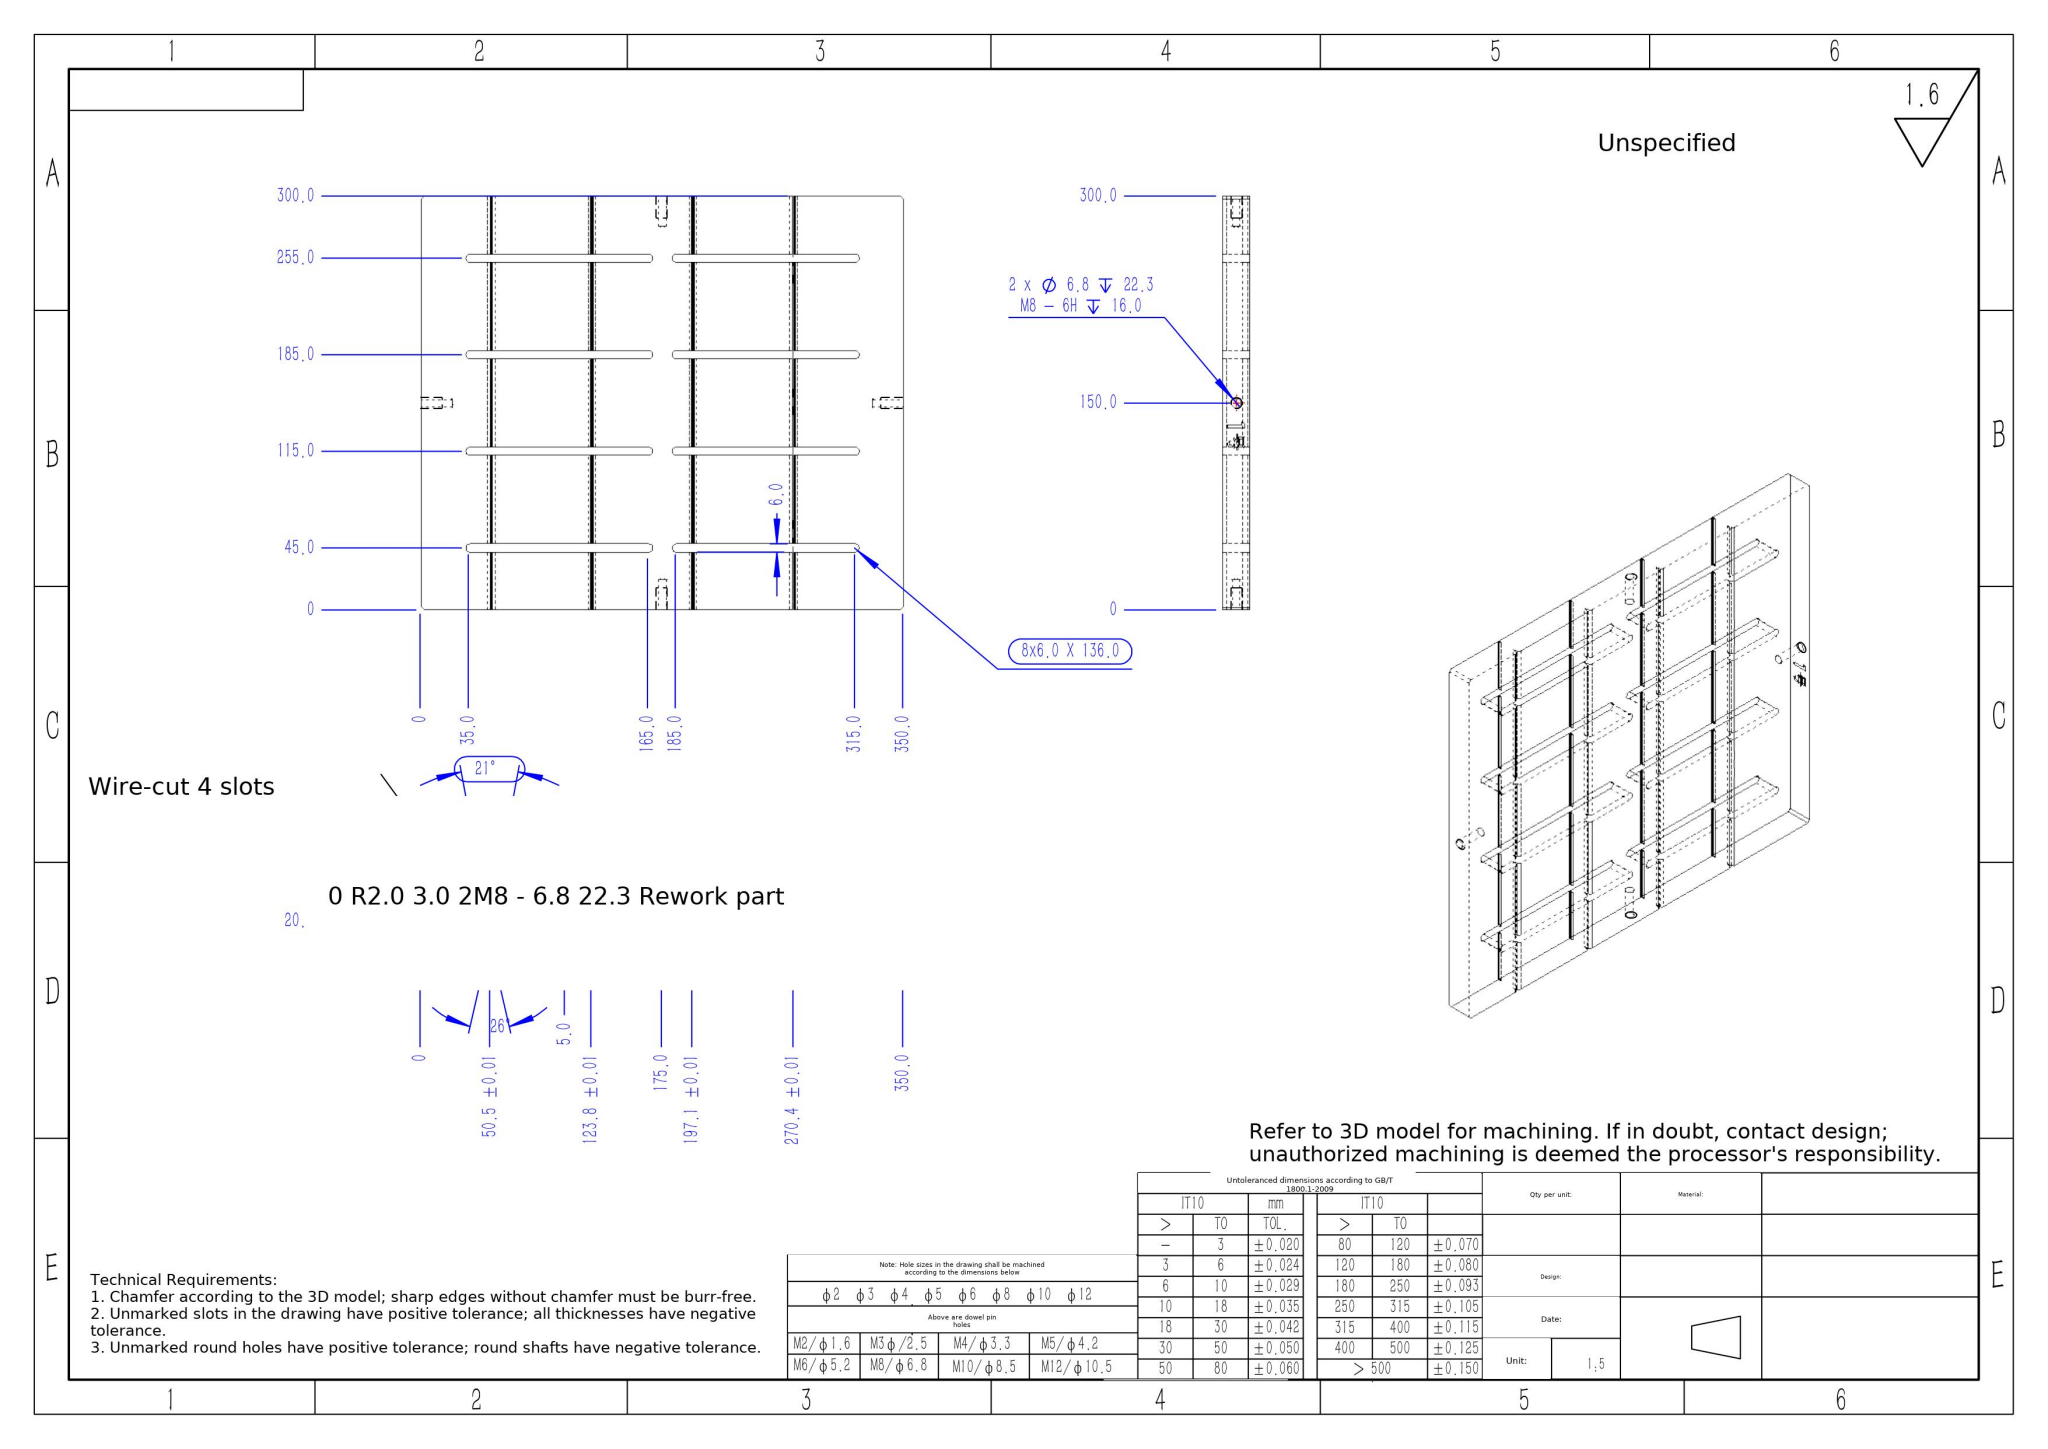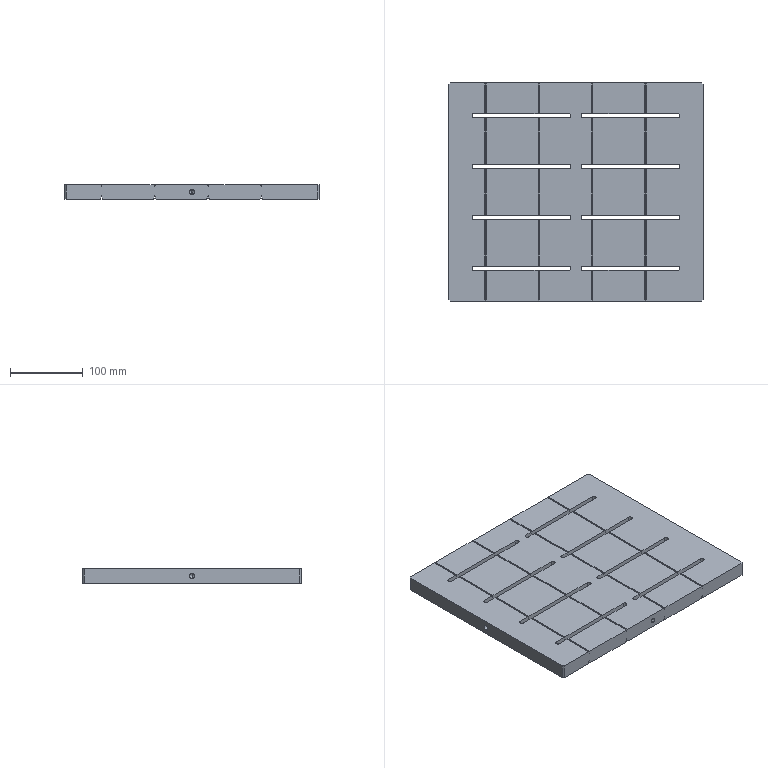Part | SolidWorks | mm | 1 solid | 297 faces | box 350 x 300 x 20 mm | volume 1957798 mm3 | plane 170 | cylinder 112 | cone 8 | spline 7 | commonest cylinder face diameters 4 x40 1 x40 6 x24 6.8 x8
build123d program:
from build123d import *

# Parameters (mm, degrees)
SKETCH1_W            = 350
SKETCH1_H            = 300
BOSS_EXTRUDE1_DEPTH  = 20
CHAMFER1_SIZE        = 2
CUT_EXTRUDE1_DEPTH   = 348.886
LPATTERN1_COUNT      = 4
LPATTERN1_PITCH      = 73.3
CUT_EXTRUDE2_DEPTH   = 0.1
SKETCH9_W            = 2.374
SKETCH9_H            = 4.924
CUT_EXTRUDE3_DEPTH   = 0.1
FILLET1_R            = 2
CUT_EXTRUDE5_DEPTH   = 161
LPATTERN4_COUNT      = 4
LPATTERN4_PITCH      = 70
MIRROR3_COPY_1_DEPTH = 161
MIRROR3_COPY_2_DEPTH = 161
MIRROR3_COPY_3_DEPTH = 161
CUT_EXTRUDE6_DEPTH   = 348.886
FILLET2_R            = 0.5
LPATTERN5_COUNT      = 4
LPATTERN5_PITCH      = 73.3
FILLET3_R            = 0.5


with BuildPart() as part:
    # Sketch1 → Boss-Extrude1 (new body)
    with BuildSketch(Plane.XY):
        Rectangle(SKETCH1_W, SKETCH1_H)
    extrude(amount=BOSS_EXTRUDE1_DEPTH)

    # Chamfer1
    chamfer1_edges = [part.edges().sort_by_distance(p)[0] for p in [
        (175, -150, 10),
        (-175, -150, 10),
        (-175, 150, 10),
        (175, 150, 10),
    ]]
    chamfer(chamfer1_edges, length=CHAMFER1_SIZE)

    # Sketch3 → Cut-Extrude1 (cut, through all)
    with BuildSketch(Plane.XZ.offset(150)):
        Polygon((96.514, 0), (94.206, 0), (95.36, 5), align=None)
    cut_extrude1 = extrude(amount=-CUT_EXTRUDE1_DEPTH, mode=Mode.SUBTRACT)

    # LPattern1: Cut-Extrude1 ×4
    with Locations(*[(-i * LPATTERN1_PITCH, 0, 0) for i in range(1, LPATTERN1_COUNT)]):
        add(cut_extrude1, mode=Mode.SUBTRACT)

    # Sketch5 → M8 Tapped Hole1 (revolve, cut)
    with BuildSketch(Plane(origin=(175, 0, 10), x_dir=(0, 0, -1), z_dir=(0, 1, 0))):
        Polygon((0, 0), (0, 24.293), (3.4, 22.25), (3.4, 0), align=None)
    m8_tapped_hole1 = revolve(axis=Axis((181.35, 0, 10), (-1, 0, 0)), mode=Mode.SUBTRACT)

    # Mirror1: M8 Tapped Hole1 across plane
    add(m8_tapped_hole1.mirror(Plane(origin=(0, 0, 0), x_dir=(0, 0, 1), z_dir=(1, 0, 0))), mode=Mode.SUBTRACT)

    # Sketch7 → M8 Tapped Hole2 (revolve, cut)
    with BuildSketch(Plane(origin=(0, 150, 10), x_dir=(0, 0, 1), z_dir=(1, 0, 0))):
        Polygon((0, 0), (0, 24.293), (3.4, 22.25), (3.4, 0), align=None)
    m8_tapped_hole2 = revolve(axis=Axis((0, 156.35, 10), (0, -1, 0)), mode=Mode.SUBTRACT)

    # Mirror2: M8 Tapped Hole2 across plane
    add(m8_tapped_hole2.mirror(Plane.ZX), mode=Mode.SUBTRACT)

    # Sketch8 → Cut-Extrude2 (cut)
    with BuildSketch(Plane(origin=(175, 0, 0), x_dir=(0, 0, -1), z_dir=(1, 0, 0))):
        Polygon((-4.143, -14.869), (-4.143, -18.198), (-16.143, -18.198), (-16.143, -16.044), (-6.143, -16.044), (-6.143, -13.583), align=None)
    extrude(amount=-CUT_EXTRUDE2_DEPTH, mode=Mode.SUBTRACT)

    # Sketch9 → Cut-Extrude3 (cut)
    # profile 1 of 2: a face of its own
    with BuildSketch(Plane(origin=(175, 0, 0), x_dir=(0, 0, -1), z_dir=(1, 0, 0))):
        with BuildLine():
            add(Edge.make_bspline(
                [(-5.014, -31.868), (-5.204, -31.868), (-5.568, -31.867), (-6.086, -31.872), (-6.553, -31.875), (-6.966, -31.881), (-7.326, -31.89), (-7.633, -31.896), (-7.887, -31.909), (-8.04, -31.918), (-8.107, -31.922)],
                knots=[0, 0, 0, 0, 1.476, 2.818, 4.025, 5.092, 6.025, 6.817, 7.476, 8, 8, 8, 8], degree=3))
            Line((-8.107, -31.922), (-8.5, -30.74))
            Line((-8.5, -30.74), (-7.969, -30.74))
            Line((-7.969, -30.74), (-7.969, -25.816))
            Line((-7.969, -25.816), (-8.383, -25.816))
            Line((-8.383, -25.816), (-8.712, -24.637))
            add(Edge.make_bspline(
                [(-8.712, -24.637), (-8.319, -24.651), (-7.538, -24.679), (-6.367, -24.693), (-5.195, -24.679), (-4.413, -24.651), (-4.02, -24.637)],
                knots=[0, 0, 0, 0, 1.004, 1.998, 2.996, 4, 4, 4, 4], degree=3))
            Line((-4.02, -24.637), (-4.445, -25.65))
            Line((-4.445, -25.65), (-4.445, -30.756))
            Line((-4.445, -30.756), (-3.866, -31.311))
            Line((-3.866, -31.311), (-4.627, -32.293))
            Line((-4.627, -32.293), (-5.014, -31.868))
        make_face()
        with Locations((-6.207, -28.278)):
            Rectangle(SKETCH9_W, SKETCH9_H, mode=Mode.SUBTRACT)
    # profile 2 of 2: a face of its own
    with BuildSketch(Plane(origin=(175, 0, 0), x_dir=(0, 0, -1), z_dir=(1, 0, 0))):
        with BuildLine():
            add(Edge.make_bspline(
                [(-11.987, -32.181), (-12.099, -32.162), (-12.317, -32.124), (-12.635, -32.066), (-12.935, -32.009), (-13.216, -31.949), (-13.48, -31.894), (-13.726, -31.838), (-13.954, -31.785), (-14.163, -31.727), (-14.356, -31.677), (-14.53, -31.623), (-14.685, -31.568), (-14.822, -31.516), (-14.944, -31.467), (-15.045, -31.415), (-15.131, -31.366), (-15.255, -31.269), (-15.411, -31.119), (-15.594, -30.919), (-15.746, -30.715), (-15.849, -30.538), (-15.919, -30.385), (-15.97, -30.25), (-16.026, -30.095), (-16.077, -29.917), (-16.135, -29.72), (-16.19, -29.502), (-16.246, -29.263), (-16.283, -29.096), (-16.302, -29.01)],
                knots=[0, 0, 0, 0, 1.605, 3.117, 4.555, 5.9, 7.17, 8.358, 9.451, 10.474, 11.41, 12.267, 13.035, 13.729, 14.341, 14.88, 15.34, 15.73, 17.095, 18.375, 19.559, 20.668, 21.257, 21.934, 22.702, 23.577, 24.536, 25.596, 26.746, 28, 28, 28, 28], degree=3))
            add(Edge.make_bspline(
                [(-16.302, -29.01), (-16.232, -28.995), (-16.09, -28.966), (-15.887, -28.863), (-15.688, -28.722), (-15.501, -28.53), (-15.315, -28.298), (-15.139, -28.02), (-14.966, -27.699), (-14.863, -27.465), (-14.81, -27.343)],
                knots=[0, 0, 0, 0, 0.7307, 1.494, 2.322, 3.232, 4.245, 5.374, 6.624, 8, 8, 8, 8], degree=3))
            Line((-14.81, -27.343), (-14.389, -27.435))
            add(Edge.make_bspline(
                [(-14.389, -27.435), (-14.423, -27.561), (-14.487, -27.804), (-14.577, -28.153), (-14.648, -28.475), (-14.708, -28.767), (-14.758, -29.029), (-14.792, -29.261), (-14.814, -29.464), (-14.817, -29.59), (-14.818, -29.649)],
                knots=[0, 0, 0, 0, 1.387, 2.666, 3.83, 4.887, 5.831, 6.663, 7.383, 8, 8, 8, 8], degree=3))
            add(Edge.make_bspline(
                [(-14.818, -29.649), (-14.816, -29.691), (-14.813, -29.781), (-14.782, -29.922), (-14.738, -30.078), (-14.701, -30.204), (-14.649, -30.291), (-14.597, -30.334), (-14.53, -30.381), (-14.44, -30.423), (-14.331, -30.469), (-14.204, -30.518), (-14.054, -30.562), (-13.885, -30.61), (-13.696, -30.659), (-13.487, -30.706), (-13.258, -30.757), (-13.008, -30.804), (-12.738, -30.854), (-12.448, -30.907), (-12.138, -30.956), (-11.925, -30.989), (-11.815, -31.007)],
                knots=[0, 0, 0, 0, 0.7003, 1.503, 2.388, 3.392, 3.681, 4.043, 4.498, 5.044, 5.695, 6.453, 7.313, 8.292, 9.369, 10.553, 11.858, 13.259, 14.782, 16.416, 18.147, 20, 20, 20, 20], degree=3))
            Line((-11.815, -31.007), (-11.815, -26.383))
            Line((-11.815, -26.383), (-12.24, -25.796))
            Line((-12.24, -25.796), (-11.342, -25.007))
            add(Edge.make_bspline(
                [(-11.342, -25.007), (-11.296, -25.072), (-11.203, -25.201), (-11.035, -25.372), (-10.845, -25.52), (-10.554, -25.686), (-10.15, -25.869), (-9.812, -26), (-9.635, -26.069)],
                knots=[0, 0, 0, 0, 0.7001, 1.398, 2.097, 2.813, 4.337, 6, 6, 6, 6], degree=3))
            Line((-9.635, -26.069), (-9.635, -23.214))
            Line((-9.635, -23.214), (-9.742, -22.655))
            Line((-9.742, -22.655), (-9.061, -22.141))
            Line((-9.061, -22.141), (-9.061, -32.461))
            Line((-9.061, -32.461), (-8.369, -33.252))
            Line((-8.369, -33.252), (-9.635, -34.416))
            Line((-9.635, -34.416), (-9.635, -27.305))
            Line((-9.635, -27.305), (-11.24, -26.614))
            Line((-11.24, -26.614), (-11.24, -31.027))
            Line((-11.24, -31.027), (-10.655, -31.71))
            Line((-10.655, -31.71), (-11.593, -32.717))
            Line((-11.593, -32.717), (-11.987, -32.181))
        make_face()
    extrude(amount=-CUT_EXTRUDE3_DEPTH, mode=Mode.SUBTRACT)

    # Fillet1
    fillet1_edges = [part.edges().sort_by_distance(p)[0] for p in [
        (96.514, 0, 0),
        (94.206, 0, 0),
        (23.214, 0, 0),
        (20.906, 0, 0),
        (-50.086, 0, 0),
        (-52.394, 0, 0),
        (-123.386, 0, 0),
        (-125.694, 0, 0),
    ]]
    fillet(fillet1_edges, radius=FILLET1_R)

    # Sketch11 → Cut-Extrude5 (cut)
    with BuildSketch(Plane(origin=(0, 0, 0), x_dir=(-1, 0, 0), z_dir=(0, 0, -1))):
        with BuildLine():
            Line((140, 102), (10, 102))
            ThreePointArc((10, 102), (7, 105), (10, 108))
            Line((10, 108), (140, 108))
            ThreePointArc((140, 108), (143, 105), (140, 102))
        make_face()
    cut_extrude5 = extrude(amount=-CUT_EXTRUDE5_DEPTH, mode=Mode.SUBTRACT)

    # LPattern4: Cut-Extrude5 ×4
    with Locations(*[(0, -i * LPATTERN4_PITCH, 0) for i in range(1, LPATTERN4_COUNT)]):
        add(cut_extrude5, mode=Mode.SUBTRACT)

    # Mirror3: Cut-Extrude5 across plane
    add(cut_extrude5.mirror(Plane(origin=(0, 0, 0), x_dir=(0, 0, 1), z_dir=(1, 0, 0))), mode=Mode.SUBTRACT)

    # Mirror3 copy 1 sketch → Mirror3 copy 1 (cut)
    with BuildSketch(Plane(origin=(0, -70, 0), x_dir=(1, 0, 0), z_dir=(0, 0, -1))):
        with BuildLine():
            Line((140, -102), (10, -102))
            ThreePointArc((10, -102), (7, -105), (10, -108))
            Line((10, -108), (140, -108))
            ThreePointArc((140, -108), (143, -105), (140, -102))
        make_face()
    extrude(amount=-MIRROR3_COPY_1_DEPTH, mode=Mode.SUBTRACT)

    # Mirror3 copy 2 sketch → Mirror3 copy 2 (cut)
    with BuildSketch(Plane(origin=(0, -140, 0), x_dir=(1, 0, 0), z_dir=(0, 0, -1))):
        with BuildLine():
            Line((140, -102), (10, -102))
            ThreePointArc((10, -102), (7, -105), (10, -108))
            Line((10, -108), (140, -108))
            ThreePointArc((140, -108), (143, -105), (140, -102))
        make_face()
    extrude(amount=-MIRROR3_COPY_2_DEPTH, mode=Mode.SUBTRACT)

    # Mirror3 copy 3 sketch → Mirror3 copy 3 (cut)
    with BuildSketch(Plane(origin=(0, -210, 0), x_dir=(1, 0, 0), z_dir=(0, 0, -1))):
        with BuildLine():
            Line((140, -102), (10, -102))
            ThreePointArc((10, -102), (7, -105), (10, -108))
            Line((10, -108), (140, -108))
            ThreePointArc((140, -108), (143, -105), (140, -102))
        make_face()
    extrude(amount=-MIRROR3_COPY_3_DEPTH, mode=Mode.SUBTRACT)

    # Sketch12 → Cut-Extrude6 (cut, through all)
    with BuildSketch(Plane(origin=(0, 150, 0), x_dir=(1, 0, 0), z_dir=(0, 1, 0))):
        Polygon((95.916, -20), (95.36, -17), (94.804, -20), align=None)
    cut_extrude6 = extrude(amount=-CUT_EXTRUDE6_DEPTH, mode=Mode.SUBTRACT)

    # Fillet2
    fillet2_edges = [part.edges().sort_by_distance(p)[0] for p in [
        (95.916, -70, 20),
        (95.916, 0, 20),
        (95.916, 70, 20),
        (95.916, 129, 20),
        (94.804, -70, 20),
        (94.804, 0, 20),
        (94.804, 70, 20),
        (94.804, 129, 20),
        (95.916, -129, 20),
        (94.804, -129, 20),
    ]]
    fillet(fillet2_edges, radius=FILLET2_R)

    # LPattern5: Cut-Extrude6 ×4
    with Locations(*[(-i * LPATTERN5_PITCH, 0, 0) for i in range(1, LPATTERN5_COUNT)]):
        add(cut_extrude6, mode=Mode.SUBTRACT)

    # Fillet3
    fillet3_edges = [part.edges().sort_by_distance(p)[0] for p in [
        (22.616, -70, 20),
        (22.616, 0, 20),
        (22.616, 70, 20),
        (22.616, 129, 20),
        (21.504, -70, 20),
        (21.504, 0, 20),
        (21.504, 70, 20),
        (21.504, 129, 20),
        (22.616, -129, 20),
        (21.504, -129, 20),
        (-50.684, 70, 20),
        (-50.684, 129, 20),
        (-50.684, -129, 20),
        (-50.684, -70, 20),
        (-50.684, 0, 20),
        (-51.796, 70, 20),
        (-51.796, 129, 20),
        (-51.796, -129, 20),
        (-51.796, -70, 20),
        (-51.796, 0, 20),
        (-123.984, 70, 20),
        (-123.984, 129, 20),
        (-123.984, -129, 20),
        (-123.984, -70, 20),
        (-123.984, 0, 20),
        (-125.096, 70, 20),
        (-125.096, 129, 20),
        (-125.096, -129, 20),
        (-125.096, -70, 20),
        (-125.096, 0, 20),
    ]]
    fillet(fillet3_edges, radius=FILLET3_R)


solid = part.part